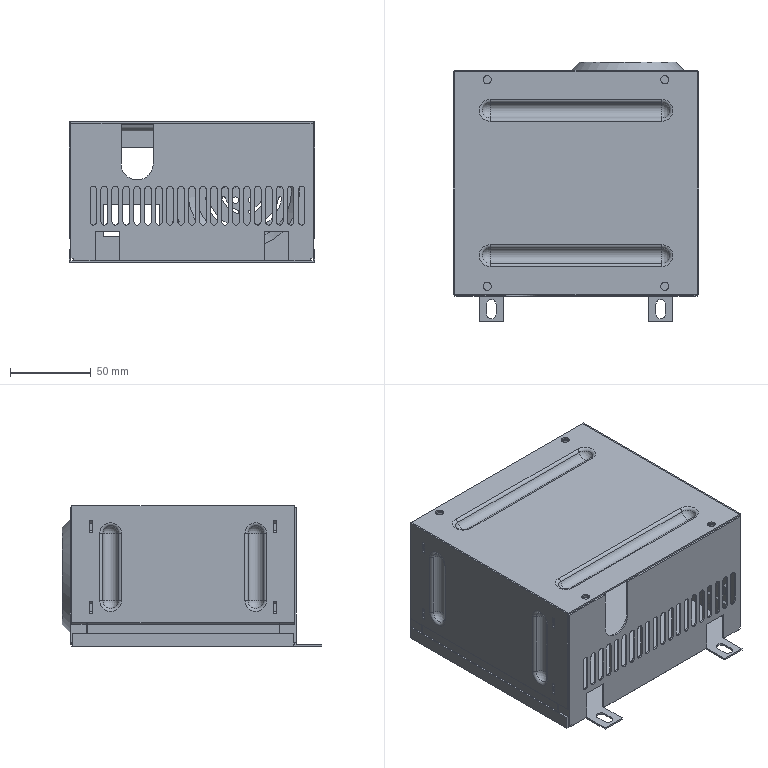Assembly | NX | mm | 6 component files | 6 solids | 464 faces | box 152 x 161 x 87 mm | volume 94319 mm3 | plane 281 | cylinder 133 | sphere 24 | torus 24 | cone 2 | commonest cylinder face diameters 4 x60 2 x28 5 x8 6 x8 10 x6 12 x6 44 x4 48 x4
Bill of materials:
unnamed part 1 | 1 |  | Thin rectangular sheet-like tray with two short upturned flanges on opposite edges and two coplanar tabs with obround slots projecting from a third edge.
unnamed part 2 | 2 |  | Rectangular thin plate with two parallel elongated raised embossments (rounded-end ribs) and an offset, jogged lip along one long edge.
unnamed part 3 | 1 |  | Flat rectangular thin plate with four corner through-holes and two long parallel stamped beads protruding from one face.
unnamed part 4 | 1 |  | Rectangular plate with short perimeter flanges, two rectangular cutouts, multiple round holes, and a raised circular dished region containing concentric arc slots and four small holes.
unnamed part 5 | 1 |  | Rectangular plate with a U-shaped slot cut down from the top edge, a row of evenly spaced vertical obround slots, two rectangular notches in the bottom edge, and a narrow top flange with two holes.
Mates:
1. touch align | side_panel 2 face | top_cover 1 face
2. touch align | side_panel 2 face | top_cover 1 face
3. center | side_panel 2 face | side_panel 2 face | top_cover 1 face | top_cover 1 face
4. touch align | side_panel 1 face | top_cover 1 face
5. touch align | side_panel 1 face | top_cover 1 face
6. touch align | side_panel 1 face | top_cover 1 face
7. concentric | rear_panel 1 edge | top_cover 1 edge
8. concentric | front_panel 1 edge | top_cover 1 edge
9. touch align | bottom_panel 1 face | rear_panel 1 face
10. center | bottom_panel 1 face | bottom_panel 1 face | side_panel 1 face | side_panel 2 face
11. touch align | bottom_panel 1 face | front_panel 1 face